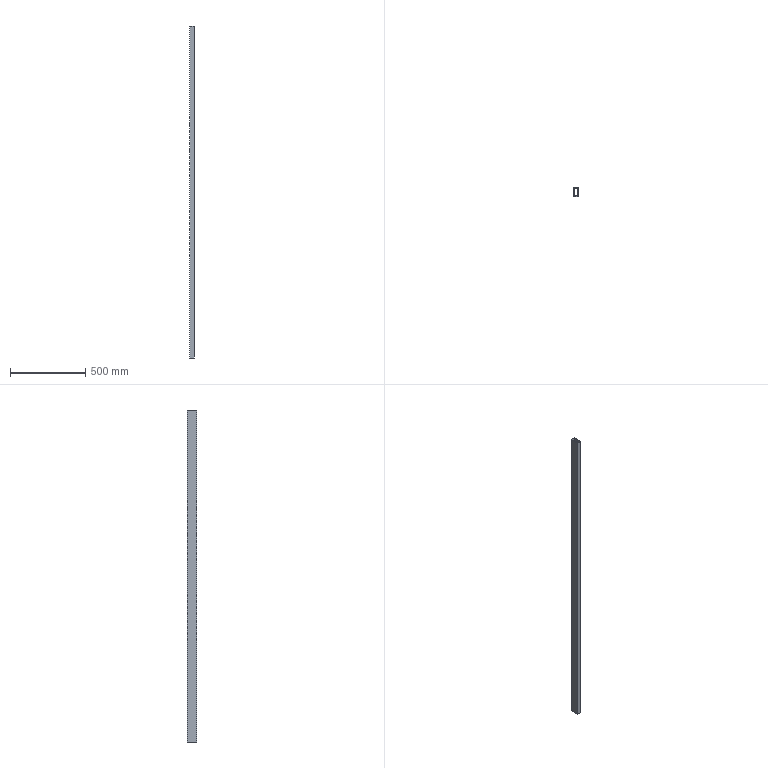Component | SolidWorks | SquareIronTube-1 | 1 solid | 18 faces | box 30 x 60 x 2200 mm | volume 756346 mm3 | plane 10 | cylinder 8 | commonest cylinder face diameters 8.5 x8
build123d program:
from build123d import *

# Parameters (mm, degrees)
SKETCH1_W           = 60
SKETCH1_H           = 30
SKETCH1_W_2         = 56
SKETCH1_H_2         = 26
BOSS_EXTRUDE1_DEPTH = 2200
SKETCH2_R           = 4.25
CUT_EXTRUDE1_DEPTH  = 10


with BuildPart() as part:
    # Sketch1 → Boss-Extrude1 (new body)
    with BuildSketch(Plane.XY):
        with Locations((30, 15)):
            Rectangle(SKETCH1_W, SKETCH1_H)
        with Locations((30, 15)):
            Rectangle(SKETCH1_W_2, SKETCH1_H_2, mode=Mode.SUBTRACT)
    extrude(amount=BOSS_EXTRUDE1_DEPTH)

    # Sketch2 → Cut-Extrude1 (cut)
    with BuildSketch(Plane(origin=(0, 30, 0), x_dir=(1, 0, 0), z_dir=(0, 1, 0))):
        with Locations(Location((30, -20, 0), (0, 0, 270))):
            Circle(SKETCH2_R)
        with Locations(Location((30, -101, 0), (0, 0, 270))):
            Circle(SKETCH2_R)
        with Locations(Location((30, -2180, 0), (0, 0, 270))):
            Circle(SKETCH2_R)
        with Locations(Location((30, -2099, 0), (0, 0, 270))):
            Circle(SKETCH2_R)
    extrude(amount=-CUT_EXTRUDE1_DEPTH, mode=Mode.SUBTRACT)


solid = part.part

# Placed as in the assembly
solid = solid.moved(Location((-151.793, 38.197, -283.936), (0, 0, -90)))
STEP:
#1=COLOUR_RGB('',0.7922,0.8196,0.9333);
#2=FILL_AREA_STYLE_COLOUR('',#1);
#3=FILL_AREA_STYLE('',(#2));
#4=SURFACE_STYLE_FILL_AREA(#3);
#5=SURFACE_SIDE_STYLE('',(#4));
#6=SURFACE_STYLE_USAGE(.BOTH.,#5);
#7=PRESENTATION_STYLE_ASSIGNMENT((#6));
#8=CARTESIAN_POINT('',(-4.874,0.3227,-10.224));
#9=VERTEX_POINT('',#8);
#10=CARTESIAN_POINT('',(-4.874,0.3227,-10.559));
#11=VERTEX_POINT('',#10);
#12=CARTESIAN_POINT('',(-4.874,0.3227,-10.391));
#13=DIRECTION('',(-1.,0.,-0.));
#14=DIRECTION('',(0.,0.,-1.));
#15=AXIS2_PLACEMENT_3D('',#12,#13,#14);
#16=CIRCLE('',#15,0.1673);
#17=EDGE_CURVE('',#9,#11,#16,.T.);
#18=ORIENTED_EDGE('',*,*,#17,.T.);
#19=CARTESIAN_POINT('',(-4.795,0.3227,-10.559));
#20=VERTEX_POINT('',#19);
#21=CARTESIAN_POINT('',(-5.189,0.3227,-10.559));
#22=DIRECTION('',(1.,-0.,0.));
#23=VECTOR('',#22,39.37);
#24=LINE('',#21,#23);
#25=EDGE_CURVE('',#11,#20,#24,.T.);
#26=ORIENTED_EDGE('',*,*,#25,.T.);
#27=CARTESIAN_POINT('',(-4.795,0.3227,-10.224));
#28=VERTEX_POINT('',#27);
#29=CARTESIAN_POINT('',(-4.795,0.3227,-10.391));
#30=DIRECTION('',(1.,-0.,0.));
#31=DIRECTION('',(0.,0.,1.));
#32=AXIS2_PLACEMENT_3D('',#29,#30,#31);
#33=CIRCLE('',#32,0.1673);
#34=EDGE_CURVE('',#20,#28,#33,.T.);
#35=ORIENTED_EDGE('',*,*,#34,.T.);
#36=CARTESIAN_POINT('',(-5.189,0.3227,-10.224));
#37=DIRECTION('',(1.,-0.,0.));
#38=VECTOR('',#37,39.37);
#39=LINE('',#36,#38);
#40=EDGE_CURVE('',#9,#28,#39,.T.);
#41=ORIENTED_EDGE('',*,*,#40,.F.);
#42=EDGE_LOOP('',(#18,#26,#35,#41));
#43=FACE_OUTER_BOUND('',#42,.T.);
#44=CARTESIAN_POINT('',(-5.189,0.3227,-10.391));
#45=DIRECTION('',(1.,-0.,0.));
#46=DIRECTION('',(0.,0.,1.));
#47=AXIS2_PLACEMENT_3D('',#44,#45,#46);
#48=CYLINDRICAL_SURFACE('',#47,0.1673);
#49=ADVANCED_FACE('',(#43),#48,.F.);
#50=CARTESIAN_POINT('',(-4.874,0.3227,71.627));
#51=VERTEX_POINT('',#50);
#52=CARTESIAN_POINT('',(-4.874,0.3227,71.292));
#53=VERTEX_POINT('',#52);
#54=CARTESIAN_POINT('',(-4.874,0.3227,71.459));
#55=DIRECTION('',(-1.,0.,-0.));
#56=DIRECTION('',(0.,0.,-1.));
#57=AXIS2_PLACEMENT_3D('',#54,#55,#56);
#58=CIRCLE('',#57,0.1673);
#59=EDGE_CURVE('',#51,#53,#58,.T.);
#60=ORIENTED_EDGE('',*,*,#59,.T.);
#61=CARTESIAN_POINT('',(-4.795,0.3227,71.292));
#62=VERTEX_POINT('',#61);
#63=CARTESIAN_POINT('',(-5.189,0.3227,71.292));
#64=DIRECTION('',(1.,-0.,0.));
#65=VECTOR('',#64,39.37);
#66=LINE('',#63,#65);
#67=EDGE_CURVE('',#53,#62,#66,.T.);
#68=ORIENTED_EDGE('',*,*,#67,.T.);
#69=CARTESIAN_POINT('',(-4.795,0.3227,71.627));
#70=VERTEX_POINT('',#69);
#71=CARTESIAN_POINT('',(-4.795,0.3227,71.459));
#72=DIRECTION('',(1.,-0.,0.));
#73=DIRECTION('',(0.,0.,1.));
#74=AXIS2_PLACEMENT_3D('',#71,#72,#73);
#75=CIRCLE('',#74,0.1673);
#76=EDGE_CURVE('',#62,#70,#75,.T.);
#77=ORIENTED_EDGE('',*,*,#76,.T.);
#78=CARTESIAN_POINT('',(-5.189,0.3227,71.627));
#79=DIRECTION('',(1.,-0.,0.));
#80=VECTOR('',#79,39.37);
#81=LINE('',#78,#80);
#82=EDGE_CURVE('',#51,#70,#81,.T.);
#83=ORIENTED_EDGE('',*,*,#82,.F.);
#84=EDGE_LOOP('',(#60,#68,#77,#83));
#85=FACE_OUTER_BOUND('',#84,.T.);
#86=CARTESIAN_POINT('',(-5.189,0.3227,71.459));
#87=DIRECTION('',(1.,-0.,0.));
#88=DIRECTION('',(0.,0.,1.));
#89=AXIS2_PLACEMENT_3D('',#86,#87,#88);
#90=CYLINDRICAL_SURFACE('',#89,0.1673);
#91=ADVANCED_FACE('',(#85),#90,.F.);
#92=CARTESIAN_POINT('',(-4.874,0.3227,74.815));
#93=VERTEX_POINT('',#92);
#94=CARTESIAN_POINT('',(-4.874,0.3227,74.481));
#95=VERTEX_POINT('',#94);
#96=CARTESIAN_POINT('',(-4.874,0.3227,74.648));
#97=DIRECTION('',(-1.,0.,-0.));
#98=DIRECTION('',(0.,0.,-1.));
#99=AXIS2_PLACEMENT_3D('',#96,#97,#98);
#100=CIRCLE('',#99,0.1673);
#101=EDGE_CURVE('',#93,#95,#100,.T.);
#102=ORIENTED_EDGE('',*,*,#101,.T.);
#103=CARTESIAN_POINT('',(-4.795,0.3227,74.481));
#104=VERTEX_POINT('',#103);
#105=CARTESIAN_POINT('',(-5.189,0.3227,74.481));
#106=DIRECTION('',(1.,-0.,0.));
#107=VECTOR('',#106,39.37);
#108=LINE('',#105,#107);
#109=EDGE_CURVE('',#95,#104,#108,.T.);
#110=ORIENTED_EDGE('',*,*,#109,.T.);
#111=CARTESIAN_POINT('',(-4.795,0.3227,74.815));
#112=VERTEX_POINT('',#111);
#113=CARTESIAN_POINT('',(-4.795,0.3227,74.648));
#114=DIRECTION('',(1.,-0.,0.));
#115=DIRECTION('',(0.,0.,1.));
#116=AXIS2_PLACEMENT_3D('',#113,#114,#115);
#117=CIRCLE('',#116,0.1673);
#118=EDGE_CURVE('',#104,#112,#117,.T.);
#119=ORIENTED_EDGE('',*,*,#118,.T.);
#120=CARTESIAN_POINT('',(-5.189,0.3227,74.815));
#121=DIRECTION('',(1.,-0.,0.));
#122=VECTOR('',#121,39.37);
#123=LINE('',#120,#122);
#124=EDGE_CURVE('',#93,#112,#123,.T.);
#125=ORIENTED_EDGE('',*,*,#124,.F.);
#126=EDGE_LOOP('',(#102,#110,#119,#125));
#127=FACE_OUTER_BOUND('',#126,.T.);
#128=CARTESIAN_POINT('',(-5.189,0.3227,74.648));
#129=DIRECTION('',(1.,-0.,0.));
#130=DIRECTION('',(0.,0.,1.));
#131=AXIS2_PLACEMENT_3D('',#128,#129,#130);
#132=CYLINDRICAL_SURFACE('',#131,0.1673);
#133=ADVANCED_FACE('',(#127),#132,.F.);
#134=CARTESIAN_POINT('',(-4.874,0.3227,-7.035));
#135=VERTEX_POINT('',#134);
#136=CARTESIAN_POINT('',(-4.874,0.3227,-7.37));
#137=VERTEX_POINT('',#136);
#138=CARTESIAN_POINT('',(-4.874,0.3227,-7.202));
#139=DIRECTION('',(-1.,0.,-0.));
#140=DIRECTION('',(0.,0.,-1.));
#141=AXIS2_PLACEMENT_3D('',#138,#139,#140);
#142=CIRCLE('',#141,0.1673);
#143=EDGE_CURVE('',#135,#137,#142,.T.);
#144=ORIENTED_EDGE('',*,*,#143,.T.);
#145=CARTESIAN_POINT('',(-4.795,0.3227,-7.37));
#146=VERTEX_POINT('',#145);
#147=CARTESIAN_POINT('',(-5.189,0.3227,-7.37));
#148=DIRECTION('',(1.,-0.,0.));
#149=VECTOR('',#148,39.37);
#150=LINE('',#147,#149);
#151=EDGE_CURVE('',#137,#146,#150,.T.);
#152=ORIENTED_EDGE('',*,*,#151,.T.);
#153=CARTESIAN_POINT('',(-4.795,0.3227,-7.035));
#154=VERTEX_POINT('',#153);
#155=CARTESIAN_POINT('',(-4.795,0.3227,-7.202));
#156=DIRECTION('',(1.,-0.,0.));
#157=DIRECTION('',(0.,0.,1.));
#158=AXIS2_PLACEMENT_3D('',#155,#156,#157);
#159=CIRCLE('',#158,0.1673);
#160=EDGE_CURVE('',#146,#154,#159,.T.);
#161=ORIENTED_EDGE('',*,*,#160,.T.);
#162=CARTESIAN_POINT('',(-5.189,0.3227,-7.035));
#163=DIRECTION('',(1.,-0.,0.));
#164=VECTOR('',#163,39.37);
#165=LINE('',#162,#164);
#166=EDGE_CURVE('',#135,#154,#165,.T.);
#167=ORIENTED_EDGE('',*,*,#166,.F.);
#168=EDGE_LOOP('',(#144,#152,#161,#167));
#169=FACE_OUTER_BOUND('',#168,.T.);
#170=CARTESIAN_POINT('',(-5.189,0.3227,-7.202));
#171=DIRECTION('',(1.,-0.,0.));
#172=DIRECTION('',(0.,0.,1.));
#173=AXIS2_PLACEMENT_3D('',#170,#171,#172);
#174=CYLINDRICAL_SURFACE('',#173,0.1673);
#175=ADVANCED_FACE('',(#169),#174,.F.);
#176=CARTESIAN_POINT('',(-5.976,1.504,75.436));
#177=VERTEX_POINT('',#176);
#178=CARTESIAN_POINT('',(-5.976,-0.8584,75.436));
#179=VERTEX_POINT('',#178);
#180=CARTESIAN_POINT('',(-5.976,-0.8584,75.436));
#181=DIRECTION('',(0.,-1.,-0.));
#182=VECTOR('',#181,39.37);
#183=LINE('',#180,#182);
#184=EDGE_CURVE('',#177,#179,#183,.T.);
#185=ORIENTED_EDGE('',*,*,#184,.T.);
#186=CARTESIAN_POINT('',(-4.795,-0.8584,75.436));
#187=VERTEX_POINT('',#186);
#188=CARTESIAN_POINT('',(-4.795,-0.8584,75.436));
#189=DIRECTION('',(1.,-0.,0.));
#190=VECTOR('',#189,39.37);
#191=LINE('',#188,#190);
#192=EDGE_CURVE('',#179,#187,#191,.T.);
#193=ORIENTED_EDGE('',*,*,#192,.T.);
#194=CARTESIAN_POINT('',(-4.795,1.504,75.436));
#195=VERTEX_POINT('',#194);
#196=CARTESIAN_POINT('',(-4.795,1.504,75.436));
#197=DIRECTION('',(0.,1.,0.));
#198=VECTOR('',#197,39.37);
#199=LINE('',#196,#198);
#200=EDGE_CURVE('',#187,#195,#199,.T.);
#201=ORIENTED_EDGE('',*,*,#200,.T.);
#202=CARTESIAN_POINT('',(-5.976,1.504,75.436));
#203=DIRECTION('',(-1.,0.,-0.));
#204=VECTOR('',#203,39.37);
#205=LINE('',#202,#204);
#206=EDGE_CURVE('',#195,#177,#205,.T.);
#207=ORIENTED_EDGE('',*,*,#206,.T.);
#208=EDGE_LOOP('',(#185,#193,#201,#207));
#209=FACE_OUTER_BOUND('',#208,.T.);
#210=CARTESIAN_POINT('',(-5.897,-0.7796,75.436));
#211=VERTEX_POINT('',#210);
#212=CARTESIAN_POINT('',(-4.874,-0.7796,75.436));
#213=VERTEX_POINT('',#212);
#214=CARTESIAN_POINT('',(-4.874,-0.7796,75.436));
#215=DIRECTION('',(1.,-0.,0.));
#216=VECTOR('',#215,39.37);
#217=LINE('',#214,#216);
#218=EDGE_CURVE('',#211,#213,#217,.T.);
#219=ORIENTED_EDGE('',*,*,#218,.F.);
#220=CARTESIAN_POINT('',(-5.897,1.425,75.436));
#221=VERTEX_POINT('',#220);
#222=CARTESIAN_POINT('',(-5.897,-0.7796,75.436));
#223=DIRECTION('',(0.,-1.,-0.));
#224=VECTOR('',#223,39.37);
#225=LINE('',#222,#224);
#226=EDGE_CURVE('',#221,#211,#225,.T.);
#227=ORIENTED_EDGE('',*,*,#226,.F.);
#228=CARTESIAN_POINT('',(-4.874,1.425,75.436));
#229=VERTEX_POINT('',#228);
#230=CARTESIAN_POINT('',(-5.897,1.425,75.436));
#231=DIRECTION('',(-1.,0.,-0.));
#232=VECTOR('',#231,39.37);
#233=LINE('',#230,#232);
#234=EDGE_CURVE('',#229,#221,#233,.T.);
#235=ORIENTED_EDGE('',*,*,#234,.F.);
#236=CARTESIAN_POINT('',(-4.874,1.425,75.436));
#237=DIRECTION('',(0.,1.,0.));
#238=VECTOR('',#237,39.37);
#239=LINE('',#236,#238);
#240=EDGE_CURVE('',#213,#229,#239,.T.);
#241=ORIENTED_EDGE('',*,*,#240,.F.);
#242=EDGE_LOOP('',(#219,#227,#235,#241));
#243=FACE_BOUND('',#242,.T.);
#244=CARTESIAN_POINT('',(-5.976,1.504,75.436));
#245=DIRECTION('',(0.,0.,-1.));
#246=DIRECTION('',(0.,1.,0.));
#247=AXIS2_PLACEMENT_3D('',#244,#245,#246);
#248=PLANE('',#247);
#249=ADVANCED_FACE('',(#209,#243),#248,.F.);
#250=CARTESIAN_POINT('',(-5.976,1.504,-11.179));
#251=VERTEX_POINT('',#250);
#252=CARTESIAN_POINT('',(-5.976,-0.8584,-11.179));
#253=VERTEX_POINT('',#252);
#254=CARTESIAN_POINT('',(-5.976,-0.8584,-11.179));
#255=DIRECTION('',(0.,-1.,-0.));
#256=VECTOR('',#255,39.37);
#257=LINE('',#254,#256);
#258=EDGE_CURVE('',#251,#253,#257,.T.);
#259=ORIENTED_EDGE('',*,*,#258,.F.);
#260=CARTESIAN_POINT('',(-4.795,1.504,-11.179));
#261=VERTEX_POINT('',#260);
#262=CARTESIAN_POINT('',(-5.976,1.504,-11.179));
#263=DIRECTION('',(-1.,0.,-0.));
#264=VECTOR('',#263,39.37);
#265=LINE('',#262,#264);
#266=EDGE_CURVE('',#261,#251,#265,.T.);
#267=ORIENTED_EDGE('',*,*,#266,.F.);
#268=CARTESIAN_POINT('',(-4.795,-0.8584,-11.179));
#269=VERTEX_POINT('',#268);
#270=CARTESIAN_POINT('',(-4.795,1.504,-11.179));
#271=DIRECTION('',(0.,1.,0.));
#272=VECTOR('',#271,39.37);
#273=LINE('',#270,#272);
#274=EDGE_CURVE('',#269,#261,#273,.T.);
#275=ORIENTED_EDGE('',*,*,#274,.F.);
#276=CARTESIAN_POINT('',(-4.795,-0.8584,-11.179));
#277=DIRECTION('',(1.,-0.,0.));
#278=VECTOR('',#277,39.37);
#279=LINE('',#276,#278);
#280=EDGE_CURVE('',#253,#269,#279,.T.);
#281=ORIENTED_EDGE('',*,*,#280,.F.);
#282=EDGE_LOOP('',(#259,#267,#275,#281));
#283=FACE_OUTER_BOUND('',#282,.T.);
#284=CARTESIAN_POINT('',(-5.897,1.425,-11.179));
#285=VERTEX_POINT('',#284);
#286=CARTESIAN_POINT('',(-5.897,-0.7796,-11.179));
#287=VERTEX_POINT('',#286);
#288=CARTESIAN_POINT('',(-5.897,-0.7796,-11.179));
#289=DIRECTION('',(0.,-1.,-0.));
#290=VECTOR('',#289,39.37);
#291=LINE('',#288,#290);
#292=EDGE_CURVE('',#285,#287,#291,.T.);
#293=ORIENTED_EDGE('',*,*,#292,.T.);
#294=CARTESIAN_POINT('',(-4.874,-0.7796,-11.179));
#295=VERTEX_POINT('',#294);
#296=CARTESIAN_POINT('',(-4.874,-0.7796,-11.179));
#297=DIRECTION('',(1.,-0.,0.));
#298=VECTOR('',#297,39.37);
#299=LINE('',#296,#298);
#300=EDGE_CURVE('',#287,#295,#299,.T.);
#301=ORIENTED_EDGE('',*,*,#300,.T.);
#302=CARTESIAN_POINT('',(-4.874,1.425,-11.179));
#303=VERTEX_POINT('',#302);
#304=CARTESIAN_POINT('',(-4.874,1.425,-11.179));
#305=DIRECTION('',(0.,1.,0.));
#306=VECTOR('',#305,39.37);
#307=LINE('',#304,#306);
#308=EDGE_CURVE('',#295,#303,#307,.T.);
#309=ORIENTED_EDGE('',*,*,#308,.T.);
#310=CARTESIAN_POINT('',(-5.897,1.425,-11.179));
#311=DIRECTION('',(-1.,0.,-0.));
#312=VECTOR('',#311,39.37);
#313=LINE('',#310,#312);
#314=EDGE_CURVE('',#303,#285,#313,.T.);
#315=ORIENTED_EDGE('',*,*,#314,.T.);
#316=EDGE_LOOP('',(#293,#301,#309,#315));
#317=FACE_BOUND('',#316,.T.);
#318=CARTESIAN_POINT('',(-5.976,1.504,-11.179));
#319=DIRECTION('',(0.,0.,-1.));
#320=DIRECTION('',(0.,1.,0.));
#321=AXIS2_PLACEMENT_3D('',#318,#319,#320);
#322=PLANE('',#321);
#323=ADVANCED_FACE('',(#283,#317),#322,.T.);
#324=ORIENTED_EDGE('',*,*,#258,.T.);
#325=CARTESIAN_POINT('',(-5.976,-0.8584,75.436));
#326=DIRECTION('',(0.,0.,-1.));
#327=VECTOR('',#326,39.37);
#328=LINE('',#325,#327);
#329=EDGE_CURVE('',#179,#253,#328,.T.);
#330=ORIENTED_EDGE('',*,*,#329,.F.);
#331=ORIENTED_EDGE('',*,*,#184,.F.);
#332=CARTESIAN_POINT('',(-5.976,1.504,75.436));
#333=DIRECTION('',(0.,0.,-1.));
#334=VECTOR('',#333,39.37);
#335=LINE('',#332,#334);
#336=EDGE_CURVE('',#177,#251,#335,.T.);
#337=ORIENTED_EDGE('',*,*,#336,.T.);
#338=EDGE_LOOP('',(#324,#330,#331,#337));
#339=FACE_OUTER_BOUND('',#338,.T.);
#340=CARTESIAN_POINT('',(-5.976,-0.8584,75.436));
#341=DIRECTION('',(1.,0.,0.));
#342=DIRECTION('',(-0.,1.,0.));
#343=AXIS2_PLACEMENT_3D('',#340,#341,#342);
#344=PLANE('',#343);
#345=ADVANCED_FACE('',(#339),#344,.F.);
#346=ORIENTED_EDGE('',*,*,#280,.T.);
#347=CARTESIAN_POINT('',(-4.795,-0.8584,75.436));
#348=DIRECTION('',(0.,0.,-1.));
#349=VECTOR('',#348,39.37);
#350=LINE('',#347,#349);
#351=EDGE_CURVE('',#187,#269,#350,.T.);
#352=ORIENTED_EDGE('',*,*,#351,.F.);
#353=ORIENTED_EDGE('',*,*,#192,.F.);
#354=ORIENTED_EDGE('',*,*,#329,.T.);
#355=EDGE_LOOP('',(#346,#352,#353,#354));
#356=FACE_OUTER_BOUND('',#355,.T.);
#357=CARTESIAN_POINT('',(-4.795,-0.8584,75.436));
#358=DIRECTION('',(0.,1.,0.));
#359=DIRECTION('',(-0.,-0.,1.));
#360=AXIS2_PLACEMENT_3D('',#357,#358,#359);
#361=PLANE('',#360);
#362=ADVANCED_FACE('',(#356),#361,.F.);
#363=CARTESIAN_POINT('',(-4.795,0.3227,-10.391));
#364=DIRECTION('',(1.,-0.,0.));
#365=DIRECTION('',(0.,0.,1.));
#366=AXIS2_PLACEMENT_3D('',#363,#364,#365);
#367=CIRCLE('',#366,0.1673);
#368=EDGE_CURVE('',#28,#20,#367,.T.);
#369=ORIENTED_EDGE('',*,*,#368,.F.);
#370=ORIENTED_EDGE('',*,*,#34,.F.);
#371=EDGE_LOOP('',(#369,#370));
#372=FACE_BOUND('',#371,.T.);
#373=CARTESIAN_POINT('',(-4.795,0.3227,71.459));
#374=DIRECTION('',(1.,-0.,0.));
#375=DIRECTION('',(0.,0.,1.));
#376=AXIS2_PLACEMENT_3D('',#373,#374,#375);
#377=CIRCLE('',#376,0.1673);
#378=EDGE_CURVE('',#70,#62,#377,.T.);
#379=ORIENTED_EDGE('',*,*,#378,.F.);
#380=ORIENTED_EDGE('',*,*,#76,.F.);
#381=EDGE_LOOP('',(#379,#380));
#382=FACE_BOUND('',#381,.T.);
#383=CARTESIAN_POINT('',(-4.795,0.3227,74.648));
#384=DIRECTION('',(1.,-0.,0.));
#385=DIRECTION('',(0.,0.,1.));
#386=AXIS2_PLACEMENT_3D('',#383,#384,#385);
#387=CIRCLE('',#386,0.1673);
#388=EDGE_CURVE('',#112,#104,#387,.T.);
#389=ORIENTED_EDGE('',*,*,#388,.F.);
#390=ORIENTED_EDGE('',*,*,#118,.F.);
#391=EDGE_LOOP('',(#389,#390));
#392=FACE_BOUND('',#391,.T.);
#393=CARTESIAN_POINT('',(-4.795,0.3227,-7.202));
#394=DIRECTION('',(1.,-0.,0.));
#395=DIRECTION('',(0.,0.,1.));
#396=AXIS2_PLACEMENT_3D('',#393,#394,#395);
#397=CIRCLE('',#396,0.1673);
#398=EDGE_CURVE('',#154,#146,#397,.T.);
#399=ORIENTED_EDGE('',*,*,#398,.F.);
#400=ORIENTED_EDGE('',*,*,#160,.F.);
#401=EDGE_LOOP('',(#399,#400));
#402=FACE_BOUND('',#401,.T.);
#403=ORIENTED_EDGE('',*,*,#274,.T.);
#404=CARTESIAN_POINT('',(-4.795,1.504,75.436));
#405=DIRECTION('',(0.,0.,-1.));
#406=VECTOR('',#405,39.37);
#407=LINE('',#404,#406);
#408=EDGE_CURVE('',#195,#261,#407,.T.);
#409=ORIENTED_EDGE('',*,*,#408,.F.);
#410=ORIENTED_EDGE('',*,*,#200,.F.);
#411=ORIENTED_EDGE('',*,*,#351,.T.);
#412=EDGE_LOOP('',(#403,#409,#410,#411));
#413=FACE_OUTER_BOUND('',#412,.T.);
#414=CARTESIAN_POINT('',(-4.795,1.504,75.436));
#415=DIRECTION('',(-1.,0.,-0.));
#416=DIRECTION('',(0.,0.,-1.));
#417=AXIS2_PLACEMENT_3D('',#414,#415,#416);
#418=PLANE('',#417);
#419=ADVANCED_FACE('',(#372,#382,#392,#402,#413),#418,.F.);
#420=ORIENTED_EDGE('',*,*,#266,.T.);
#421=ORIENTED_EDGE('',*,*,#336,.F.);
#422=ORIENTED_EDGE('',*,*,#206,.F.);
#423=ORIENTED_EDGE('',*,*,#408,.T.);
#424=EDGE_LOOP('',(#420,#421,#422,#423));
#425=FACE_OUTER_BOUND('',#424,.T.);
#426=CARTESIAN_POINT('',(-5.976,1.504,75.436));
#427=DIRECTION('',(-0.,-1.,-0.));
#428=DIRECTION('',(0.,0.,-1.));
#429=AXIS2_PLACEMENT_3D('',#426,#427,#428);
#430=PLANE('',#429);
#431=ADVANCED_FACE('',(#425),#430,.F.);
#432=ORIENTED_EDGE('',*,*,#300,.F.);
#433=CARTESIAN_POINT('',(-5.897,-0.7796,75.436));
#434=DIRECTION('',(0.,0.,-1.));
#435=VECTOR('',#434,39.37);
#436=LINE('',#433,#435);
#437=EDGE_CURVE('',#211,#287,#436,.T.);
#438=ORIENTED_EDGE('',*,*,#437,.F.);
#439=ORIENTED_EDGE('',*,*,#218,.T.);
#440=CARTESIAN_POINT('',(-4.874,-0.7796,75.436));
#441=DIRECTION('',(0.,0.,-1.));
#442=VECTOR('',#441,39.37);
#443=LINE('',#440,#442);
#444=EDGE_CURVE('',#213,#295,#443,.T.);
#445=ORIENTED_EDGE('',*,*,#444,.T.);
#446=EDGE_LOOP('',(#432,#438,#439,#445));
#447=FACE_OUTER_BOUND('',#446,.T.);
#448=CARTESIAN_POINT('',(-4.874,-0.7796,75.436));
#449=DIRECTION('',(0.,1.,0.));
#450=DIRECTION('',(-0.,-0.,1.));
#451=AXIS2_PLACEMENT_3D('',#448,#449,#450);
#452=PLANE('',#451);
#453=ADVANCED_FACE('',(#447),#452,.T.);
#454=ORIENTED_EDGE('',*,*,#17,.F.);
#455=CARTESIAN_POINT('',(-4.874,0.3227,-10.391));
#456=DIRECTION('',(-1.,0.,-0.));
#457=DIRECTION('',(0.,0.,-1.));
#458=AXIS2_PLACEMENT_3D('',#455,#456,#457);
#459=CIRCLE('',#458,0.1673);
#460=EDGE_CURVE('',#11,#9,#459,.T.);
#461=ORIENTED_EDGE('',*,*,#460,.F.);
#462=EDGE_LOOP('',(#454,#461));
#463=FACE_BOUND('',#462,.T.);
#464=ORIENTED_EDGE('',*,*,#59,.F.);
#465=CARTESIAN_POINT('',(-4.874,0.3227,71.459));
#466=DIRECTION('',(-1.,0.,-0.));
#467=DIRECTION('',(0.,0.,-1.));
#468=AXIS2_PLACEMENT_3D('',#465,#466,#467);
#469=CIRCLE('',#468,0.1673);
#470=EDGE_CURVE('',#53,#51,#469,.T.);
#471=ORIENTED_EDGE('',*,*,#470,.F.);
#472=EDGE_LOOP('',(#464,#471));
#473=FACE_BOUND('',#472,.T.);
#474=ORIENTED_EDGE('',*,*,#101,.F.);
#475=CARTESIAN_POINT('',(-4.874,0.3227,74.648));
#476=DIRECTION('',(-1.,0.,-0.));
#477=DIRECTION('',(0.,0.,-1.));
#478=AXIS2_PLACEMENT_3D('',#475,#476,#477);
#479=CIRCLE('',#478,0.1673);
#480=EDGE_CURVE('',#95,#93,#479,.T.);
#481=ORIENTED_EDGE('',*,*,#480,.F.);
#482=EDGE_LOOP('',(#474,#481));
#483=FACE_BOUND('',#482,.T.);
#484=ORIENTED_EDGE('',*,*,#143,.F.);
#485=CARTESIAN_POINT('',(-4.874,0.3227,-7.202));
#486=DIRECTION('',(-1.,0.,-0.));
#487=DIRECTION('',(0.,0.,-1.));
#488=AXIS2_PLACEMENT_3D('',#485,#486,#487);
#489=CIRCLE('',#488,0.1673);
#490=EDGE_CURVE('',#137,#135,#489,.T.);
#491=ORIENTED_EDGE('',*,*,#490,.F.);
#492=EDGE_LOOP('',(#484,#491));
#493=FACE_BOUND('',#492,.T.);
#494=ORIENTED_EDGE('',*,*,#308,.F.);
#495=ORIENTED_EDGE('',*,*,#444,.F.);
#496=ORIENTED_EDGE('',*,*,#240,.T.);
#497=CARTESIAN_POINT('',(-4.874,1.425,75.436));
#498=DIRECTION('',(0.,0.,-1.));
#499=VECTOR('',#498,39.37);
#500=LINE('',#497,#499);
#501=EDGE_CURVE('',#229,#303,#500,.T.);
#502=ORIENTED_EDGE('',*,*,#501,.T.);
#503=EDGE_LOOP('',(#494,#495,#496,#502));
#504=FACE_OUTER_BOUND('',#503,.T.);
#505=CARTESIAN_POINT('',(-4.874,1.425,75.436));
#506=DIRECTION('',(-1.,0.,-0.));
#507=DIRECTION('',(0.,0.,-1.));
#508=AXIS2_PLACEMENT_3D('',#505,#506,#507);
#509=PLANE('',#508);
#510=ADVANCED_FACE('',(#463,#473,#483,#493,#504),#509,.T.);
#511=ORIENTED_EDGE('',*,*,#314,.F.);
#512=ORIENTED_EDGE('',*,*,#501,.F.);
#513=ORIENTED_EDGE('',*,*,#234,.T.);
#514=CARTESIAN_POINT('',(-5.897,1.425,75.436));
#515=DIRECTION('',(0.,0.,-1.));
#516=VECTOR('',#515,39.37);
#517=LINE('',#514,#516);
#518=EDGE_CURVE('',#221,#285,#517,.T.);
#519=ORIENTED_EDGE('',*,*,#518,.T.);
#520=EDGE_LOOP('',(#511,#512,#513,#519));
#521=FACE_OUTER_BOUND('',#520,.T.);
#522=CARTESIAN_POINT('',(-5.897,1.425,75.436));
#523=DIRECTION('',(-0.,-1.,-0.));
#524=DIRECTION('',(0.,0.,-1.));
#525=AXIS2_PLACEMENT_3D('',#522,#523,#524);
#526=PLANE('',#525);
#527=ADVANCED_FACE('',(#521),#526,.T.);
#528=ORIENTED_EDGE('',*,*,#292,.F.);
#529=ORIENTED_EDGE('',*,*,#518,.F.);
#530=ORIENTED_EDGE('',*,*,#226,.T.);
#531=ORIENTED_EDGE('',*,*,#437,.T.);
#532=EDGE_LOOP('',(#528,#529,#530,#531));
#533=FACE_OUTER_BOUND('',#532,.T.);
#534=CARTESIAN_POINT('',(-5.897,-0.7796,75.436));
#535=DIRECTION('',(1.,0.,0.));
#536=DIRECTION('',(-0.,1.,0.));
#537=AXIS2_PLACEMENT_3D('',#534,#535,#536);
#538=PLANE('',#537);
#539=ADVANCED_FACE('',(#533),#538,.T.);
#540=ORIENTED_EDGE('',*,*,#151,.F.);
#541=ORIENTED_EDGE('',*,*,#490,.T.);
#542=ORIENTED_EDGE('',*,*,#166,.T.);
#543=ORIENTED_EDGE('',*,*,#398,.T.);
#544=EDGE_LOOP('',(#540,#541,#542,#543));
#545=FACE_OUTER_BOUND('',#544,.T.);
#546=CARTESIAN_POINT('',(-5.189,0.3227,-7.202));
#547=DIRECTION('',(1.,-0.,0.));
#548=DIRECTION('',(0.,0.,1.));
#549=AXIS2_PLACEMENT_3D('',#546,#547,#548);
#550=CYLINDRICAL_SURFACE('',#549,0.1673);
#551=ADVANCED_FACE('',(#545),#550,.F.);
#552=ORIENTED_EDGE('',*,*,#109,.F.);
#553=ORIENTED_EDGE('',*,*,#480,.T.);
#554=ORIENTED_EDGE('',*,*,#124,.T.);
#555=ORIENTED_EDGE('',*,*,#388,.T.);
#556=EDGE_LOOP('',(#552,#553,#554,#555));
#557=FACE_OUTER_BOUND('',#556,.T.);
#558=CARTESIAN_POINT('',(-5.189,0.3227,74.648));
#559=DIRECTION('',(1.,-0.,0.));
#560=DIRECTION('',(0.,0.,1.));
#561=AXIS2_PLACEMENT_3D('',#558,#559,#560);
#562=CYLINDRICAL_SURFACE('',#561,0.1673);
#563=ADVANCED_FACE('',(#557),#562,.F.);
#564=ORIENTED_EDGE('',*,*,#67,.F.);
#565=ORIENTED_EDGE('',*,*,#470,.T.);
#566=ORIENTED_EDGE('',*,*,#82,.T.);
#567=ORIENTED_EDGE('',*,*,#378,.T.);
#568=EDGE_LOOP('',(#564,#565,#566,#567));
#569=FACE_OUTER_BOUND('',#568,.T.);
#570=CARTESIAN_POINT('',(-5.189,0.3227,71.459));
#571=DIRECTION('',(1.,-0.,0.));
#572=DIRECTION('',(0.,0.,1.));
#573=AXIS2_PLACEMENT_3D('',#570,#571,#572);
#574=CYLINDRICAL_SURFACE('',#573,0.1673);
#575=ADVANCED_FACE('',(#569),#574,.F.);
#576=ORIENTED_EDGE('',*,*,#25,.F.);
#577=ORIENTED_EDGE('',*,*,#460,.T.);
#578=ORIENTED_EDGE('',*,*,#40,.T.);
#579=ORIENTED_EDGE('',*,*,#368,.T.);
#580=EDGE_LOOP('',(#576,#577,#578,#579));
#581=FACE_OUTER_BOUND('',#580,.T.);
#582=CARTESIAN_POINT('',(-5.189,0.3227,-10.391));
#583=DIRECTION('',(1.,-0.,0.));
#584=DIRECTION('',(0.,0.,1.));
#585=AXIS2_PLACEMENT_3D('',#582,#583,#584);
#586=CYLINDRICAL_SURFACE('',#585,0.1673);
#587=ADVANCED_FACE('',(#581),#586,.F.);
#588=CLOSED_SHELL('',(#49,#91,#133,#175,#249,#323,#345,#362,#419,#431,#453,#510,#527,#539,#551,#563,#575,#587));
#589=MANIFOLD_SOLID_BREP('',#588);
#590=STYLED_ITEM('',(#7),#589);
#591=PRESENTATION_LAYER_ASSIGNMENT('','',(#590));
#592=CARTESIAN_POINT('',(0.,0.,0.));
#593=DIRECTION('',(0.,0.,1.));
#594=DIRECTION('',(1.,0.,0.));
#595=AXIS2_PLACEMENT_3D('',#592,#593,#594);
#596=(LENGTH_UNIT()NAMED_UNIT(*)SI_UNIT($,.METRE.));
#597=LENGTH_MEASURE_WITH_UNIT(LENGTH_MEASURE(0.0254),#596);
#598=DIMENSIONAL_EXPONENTS(1.,0.,0.,0.,0.,0.,0.);
#599=(CONVERSION_BASED_UNIT('',#597)LENGTH_UNIT()NAMED_UNIT(#598));
#600=UNCERTAINTY_MEASURE_WITH_UNIT(LENGTH_MEASURE(0.00001),#599,'','');
#601=(NAMED_UNIT(*)PLANE_ANGLE_UNIT()SI_UNIT($,.RADIAN.));
#602=(NAMED_UNIT(*)SI_UNIT($,.STERADIAN.)SOLID_ANGLE_UNIT());
#603=(GEOMETRIC_REPRESENTATION_CONTEXT(3)GLOBAL_UNCERTAINTY_ASSIGNED_CONTEXT((#600))GLOBAL_UNIT_ASSIGNED_CONTEXT((#599,#601,#602))REPRESENTATION_CONTEXT('',''));
#604=ADVANCED_BREP_SHAPE_REPRESENTATION('',(#589,#595),#603);
#605=(LENGTH_UNIT()NAMED_UNIT(*)SI_UNIT($,.METRE.));
#606=LENGTH_MEASURE_WITH_UNIT(LENGTH_MEASURE(0.0254),#605);
#607=DIMENSIONAL_EXPONENTS(1.,0.,0.,0.,0.,0.,0.);
#608=(CONVERSION_BASED_UNIT('',#606)LENGTH_UNIT()NAMED_UNIT(#607));
#609=UNCERTAINTY_MEASURE_WITH_UNIT(LENGTH_MEASURE(0.00001),#608,'','');
#610=(NAMED_UNIT(*)PLANE_ANGLE_UNIT()SI_UNIT($,.RADIAN.));
#611=(NAMED_UNIT(*)SI_UNIT($,.STERADIAN.)SOLID_ANGLE_UNIT());
#612=(GEOMETRIC_REPRESENTATION_CONTEXT(3)GLOBAL_UNCERTAINTY_ASSIGNED_CONTEXT((#609))GLOBAL_UNIT_ASSIGNED_CONTEXT((#608,#610,#611))REPRESENTATION_CONTEXT('',''));
#613=MECHANICAL_DESIGN_GEOMETRIC_PRESENTATION_REPRESENTATION('',(#590),#612);